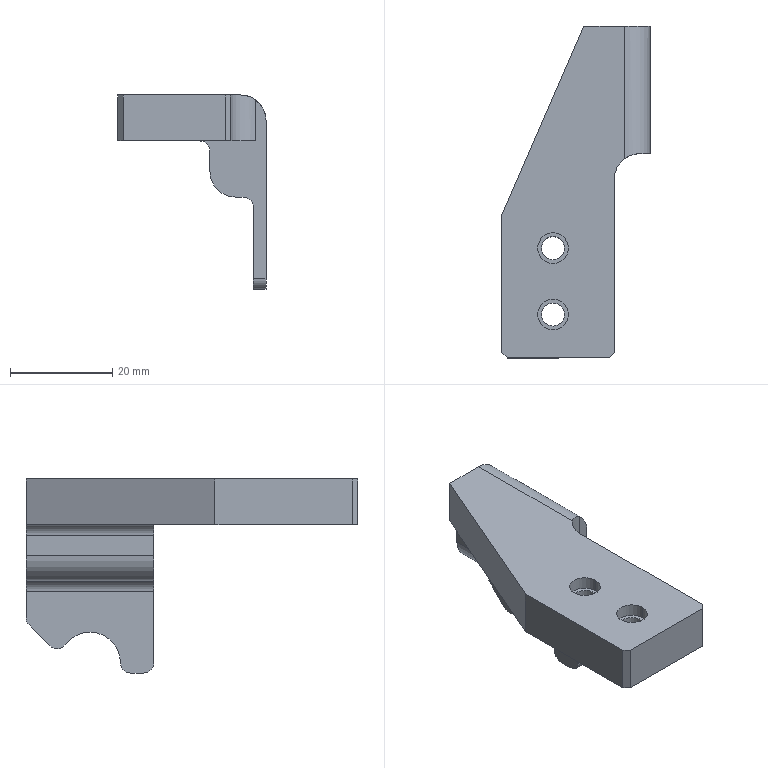Component | SolidWorks | GripperA3-2-1_AX.B92.SA.7371.37-1 | 1 solid | 43 faces | volume 14802 mm3 | cylinder 23 | plane 20 | commonest cylinder face diameters 4 x6 6 x4 8 x4 4.5 x4 10 x3 12 x2 | material 40Cr